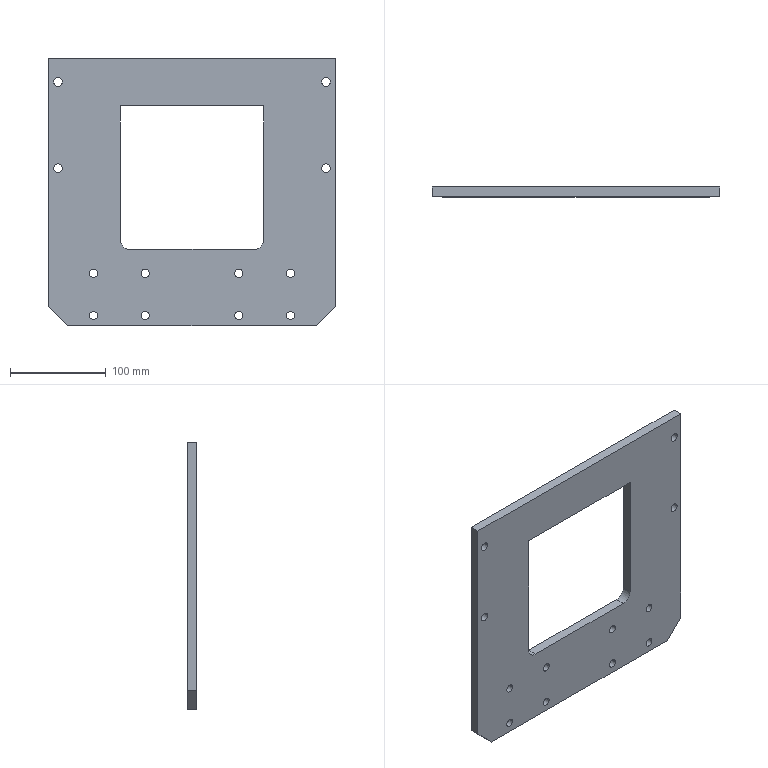Component | SolidWorks | DoubleFilmTransport-1_FilmPullingFixingBase-1 | 1 solid | 44 faces | box 300 x 10 x 280 mm | volume 603544 mm3 | cylinder 28 | plane 12 | cone 4 | commonest cylinder face diameters 8.5 x16 9 x8 6.8 x2 20 x2
build123d program:
from build123d import *

# Parameters (mm, degrees)
SKETCH1_W                      = 300
SKETCH1_H                      = 280
BOSS_EXTRUDE1_DEPTH            = 10
SKETCH2_W                      = 150
SKETCH2_H                      = 150
CUT_EXTRUDE1_DEPTH             = 206.426
F_8_5_8_5_DIAMETER_HOLE1_D     = 8.5
F_9_0_9_DIAMETER_HOLE1_D       = 9
F_6_8_6_8_DIAMETER_HOLE1_D     = 6.8
F_6_8_6_8_DIAMETER_HOLE1_DEPTH = 21.25
F_6_8_6_8_DIAMETER_HOLE1_TIP   = 2.043
CHAMFER1_SIZE                  = 20
CHAMFER2_SIZE                  = 0.625
FILLET1_R                      = 10


with BuildPart() as part:
    # Sketch1 → Boss-Extrude1 (new body)
    with BuildSketch(Plane.XY.offset(5)):
        Rectangle(SKETCH1_W, SKETCH1_H)
    extrude(amount=-BOSS_EXTRUDE1_DEPTH)

    # Sketch2 → Cut-Extrude1 (cut, through all)
    with BuildSketch(Plane(origin=(0, 0, -5), x_dir=(-1, 0, 0), z_dir=(0, 0, -1))):
        with Locations((0, 15)):
            Rectangle(SKETCH2_W, SKETCH2_H)
    extrude(amount=-CUT_EXTRUDE1_DEPTH, mode=Mode.SUBTRACT)

    # 8.5 _8.5_ Diameter Hole1 (through all)
    with Locations(Plane(origin=(0, 0, -5), x_dir=(-1, 0, 0), z_dir=(0, 0, -1))):
        with Locations((-49, -85), (-103, -129), (49, -129), (49, -85), (103, -85), (103, -129), (-103, -85), (-49, -129)):
            Hole(F_8_5_8_5_DIAMETER_HOLE1_D / 2)

    # 9.0 _9_ Diameter Hole1 (through all)
    with Locations(Plane(origin=(0, 0, -5), x_dir=(-1, 0, 0), z_dir=(0, 0, -1))):
        with Locations((-140, 115), (140, 25), (140, 115), (-140, 25)):
            Hole(F_9_0_9_DIAMETER_HOLE1_D / 2)

    # 6.8 _6.8_ Diameter Hole1
    with Locations(Plane(origin=(150, 0, 0), x_dir=(0, 0, -1), z_dir=(1, 0, 0))):
        with Locations((0, -25)):
            Hole(F_6_8_6_8_DIAMETER_HOLE1_D / 2, depth=F_6_8_6_8_DIAMETER_HOLE1_DEPTH)
            with Locations((0, 0, -(F_6_8_6_8_DIAMETER_HOLE1_DEPTH + F_6_8_6_8_DIAMETER_HOLE1_TIP / 2))):  # 118° drill point
                Cone(0, F_6_8_6_8_DIAMETER_HOLE1_D / 2, F_6_8_6_8_DIAMETER_HOLE1_TIP, mode=Mode.SUBTRACT)

    # Chamfer1
    chamfer1_edges = [part.edges().sort_by_distance(p)[0] for p in [
        (150, -140, 0),
        (-150, -140, 0),
    ]]
    chamfer(chamfer1_edges, length=CHAMFER1_SIZE)

    # Chamfer2
    chamfer2_edges = [part.edges().sort_by_distance(p)[0] for p in [
        (150, -25, -3.4),
    ]]
    chamfer(chamfer2_edges, length=CHAMFER2_SIZE)

    # Fillet1
    fillet1_edges = [part.edges().sort_by_distance(p)[0] for p in [
        (-75, -60, 0),
        (75, -60, 0),
    ]]
    fillet(fillet1_edges, radius=FILLET1_R)


solid = part.part

# Placed as in the assembly
solid = solid.moved(Location((-298.746, 38.373, -171.5), (90, 0, 0)))